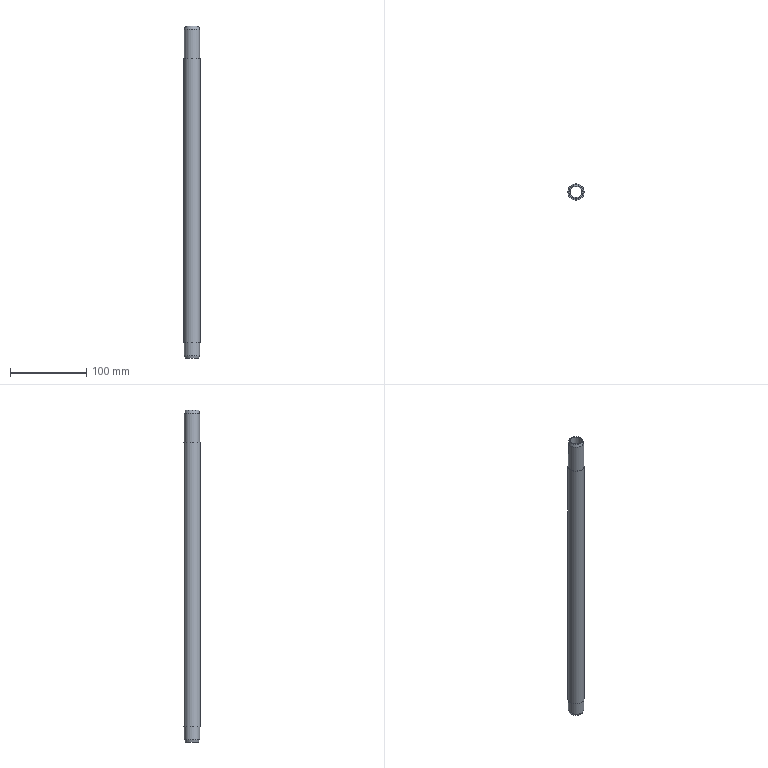Component | NX | CH3404_8-3 | 1 solid | 10 faces | box 21.3 x 21.3 x 435 mm | volume 75305 mm3 | plane 4 | cylinder 4 | cone 2 | commonest cylinder face diameters 20 x2 21.3 x1 15 x1
STEP:
#1=CARTESIAN_POINT('',(0.,0.,0.));
#2=DIRECTION('',(0.,0.,1.));
#3=DIRECTION('',(1.,0.,0.));
#4=AXIS2_PLACEMENT_3D('',#1,#2,#3);
#5=CARTESIAN_POINT('',(-10.65,0.,493.));
#6=VERTEX_POINT('',#5);
#7=CARTESIAN_POINT('',(0.,0.,493.));
#8=DIRECTION('',(0.,0.,-1.));
#9=DIRECTION('',(-1.,0.,0.));
#10=AXIS2_PLACEMENT_3D('',#7,#8,#9);
#11=CIRCLE('',#10,10.65);
#12=CARTESIAN_POINT('',(0.,-10.,493.));
#13=DIRECTION('',(0.,0.,-1.));
#14=DIRECTION('',(-1.,0.,0.));
#15=AXIS2_PLACEMENT_3D('',#12,#13,#14);
#16=PLANE('',#15);
#17=CARTESIAN_POINT('',(0.,10.));
#18=DIRECTION('',(1.,0.));
#19=AXIS2_PLACEMENT_2D('',#17,#18);
#20=CIRCLE('',#19,10.65);
#21=(GEOMETRIC_REPRESENTATION_CONTEXT(2)PARAMETRIC_REPRESENTATION_CONTEXT()REPRESENTATION_CONTEXT('',''));
#22=DEFINITIONAL_REPRESENTATION('',(#20),#21);
#23=PCURVE('',#16,#22);
#24=CARTESIAN_POINT('',(0.,0.,100.));
#25=DIRECTION('',(0.,0.,-1.));
#26=DIRECTION('',(-1.,0.,0.));
#27=AXIS2_PLACEMENT_3D('',#24,#25,#26);
#28=CYLINDRICAL_SURFACE('',#27,10.65);
#29=CARTESIAN_POINT('',(0.,-393.));
#30=DIRECTION('',(1.,0.));
#31=VECTOR('',#30,1.);
#32=LINE('',#29,#31);
#33=(GEOMETRIC_REPRESENTATION_CONTEXT(2)PARAMETRIC_REPRESENTATION_CONTEXT()REPRESENTATION_CONTEXT('',''));
#34=DEFINITIONAL_REPRESENTATION('',(#32),#33);
#35=PCURVE('',#28,#34);
#36=SURFACE_CURVE('',#11,(#23,#35),.PCURVE_S1.);
#37=EDGE_CURVE('',#6,#6,#36,.T.);
#38=ORIENTED_EDGE('',*,*,#37,.F.);
#39=EDGE_LOOP('',(#38));
#40=FACE_BOUND('',#39,.T.);
#41=CARTESIAN_POINT('',(-10.,0.,493.));
#42=VERTEX_POINT('',#41);
#43=CARTESIAN_POINT('',(0.,0.,493.));
#44=DIRECTION('',(0.,0.,-1.));
#45=DIRECTION('',(-1.,0.,0.));
#46=AXIS2_PLACEMENT_3D('',#43,#44,#45);
#47=CIRCLE('',#46,10.);
#48=CARTESIAN_POINT('',(0.,10.));
#49=DIRECTION('',(1.,0.));
#50=AXIS2_PLACEMENT_2D('',#48,#49);
#51=CIRCLE('',#50,10.);
#52=(GEOMETRIC_REPRESENTATION_CONTEXT(2)PARAMETRIC_REPRESENTATION_CONTEXT()REPRESENTATION_CONTEXT('',''));
#53=DEFINITIONAL_REPRESENTATION('',(#51),#52);
#54=PCURVE('',#16,#53);
#55=CARTESIAN_POINT('',(0.,0.,100.));
#56=DIRECTION('',(0.,0.,-1.));
#57=DIRECTION('',(-1.,0.,0.));
#58=AXIS2_PLACEMENT_3D('',#55,#56,#57);
#59=CYLINDRICAL_SURFACE('',#58,10.);
#60=CARTESIAN_POINT('',(0.,-393.));
#61=DIRECTION('',(1.,0.));
#62=VECTOR('',#61,1.);
#63=LINE('',#60,#62);
#64=(GEOMETRIC_REPRESENTATION_CONTEXT(2)PARAMETRIC_REPRESENTATION_CONTEXT()REPRESENTATION_CONTEXT('',''));
#65=DEFINITIONAL_REPRESENTATION('',(#63),#64);
#66=PCURVE('',#59,#65);
#67=SURFACE_CURVE('',#47,(#54,#66),.PCURVE_S1.);
#68=EDGE_CURVE('',#42,#42,#67,.T.);
#69=ORIENTED_EDGE('',*,*,#68,.T.);
#70=EDGE_LOOP('',(#69));
#71=FACE_BOUND('',#70,.T.);
#72=ADVANCED_FACE('',(#40,#71),#16,.F.);
#73=CARTESIAN_POINT('',(-10.65,0.,120.));
#74=VERTEX_POINT('',#73);
#75=CARTESIAN_POINT('',(0.,0.,120.));
#76=DIRECTION('',(0.,0.,-1.));
#77=DIRECTION('',(-1.,0.,0.));
#78=AXIS2_PLACEMENT_3D('',#75,#76,#77);
#79=CIRCLE('',#78,10.65);
#80=CARTESIAN_POINT('',(0.,-20.));
#81=DIRECTION('',(1.,0.));
#82=VECTOR('',#81,1.);
#83=LINE('',#80,#82);
#84=(GEOMETRIC_REPRESENTATION_CONTEXT(2)PARAMETRIC_REPRESENTATION_CONTEXT()REPRESENTATION_CONTEXT('',''));
#85=DEFINITIONAL_REPRESENTATION('',(#83),#84);
#86=PCURVE('',#28,#85);
#87=CARTESIAN_POINT('',(0.,-10.65,120.));
#88=DIRECTION('',(0.,0.,1.));
#89=DIRECTION('',(1.,0.,0.));
#90=AXIS2_PLACEMENT_3D('',#87,#88,#89);
#91=PLANE('',#90);
#92=CARTESIAN_POINT('',(-10.65,10.65));
#93=CARTESIAN_POINT('',(-10.65,29.096));
#94=CARTESIAN_POINT('',(5.325,19.873));
#95=CARTESIAN_POINT('',(21.3,10.65));
#96=CARTESIAN_POINT('',(5.325,1.427));
#97=CARTESIAN_POINT('',(-10.65,-7.796));
#98=CARTESIAN_POINT('',(-10.65,10.65));
#99=(BOUNDED_CURVE()B_SPLINE_CURVE(2,(#92,#93,#94,#95,#96,#97,#98),.UNSPECIFIED.,.T.,.F.)B_SPLINE_CURVE_WITH_KNOTS((1,2,2,2,2,1),(-2.094,0.,2.094,4.189,6.283,8.378),.UNSPECIFIED.)CURVE()GEOMETRIC_REPRESENTATION_ITEM()RATIONAL_B_SPLINE_CURVE((1.,0.5,1.,0.5,1.,0.5,1.))REPRESENTATION_ITEM(''));
#100=(GEOMETRIC_REPRESENTATION_CONTEXT(2)PARAMETRIC_REPRESENTATION_CONTEXT()REPRESENTATION_CONTEXT('',''));
#101=DEFINITIONAL_REPRESENTATION('',(#99),#100);
#102=PCURVE('',#91,#101);
#103=SURFACE_CURVE('',#79,(#86,#102),.PCURVE_S1.);
#104=EDGE_CURVE('',#74,#74,#103,.T.);
#105=ORIENTED_EDGE('',*,*,#104,.F.);
#106=CARTESIAN_POINT('',(-10.65,-0.,493.));
#107=CARTESIAN_POINT('',(-10.65,-0.,120.));
#108=B_SPLINE_CURVE_WITH_KNOTS('',1,(#106,#107),.UNSPECIFIED.,.F.,.F.,(2,2),(-393.,-20.),.PIECEWISE_BEZIER_KNOTS.);
#109=CARTESIAN_POINT('',(0.,0.));
#110=DIRECTION('',(0.,1.));
#111=VECTOR('',#110,1.);
#112=LINE('',#109,#111);
#113=(GEOMETRIC_REPRESENTATION_CONTEXT(2)PARAMETRIC_REPRESENTATION_CONTEXT()REPRESENTATION_CONTEXT('',''));
#114=DEFINITIONAL_REPRESENTATION('',(#112),#113);
#115=PCURVE('',#28,#114);
#116=CARTESIAN_POINT('',(6.283,0.));
#117=DIRECTION('',(0.,1.));
#118=VECTOR('',#117,1.);
#119=LINE('',#116,#118);
#120=(GEOMETRIC_REPRESENTATION_CONTEXT(2)PARAMETRIC_REPRESENTATION_CONTEXT()REPRESENTATION_CONTEXT('',''));
#121=DEFINITIONAL_REPRESENTATION('',(#119),#120);
#122=PCURVE('',#28,#121);
#123=SEAM_CURVE('',#108,(#115,#122),.PCURVE_S1.);
#124=EDGE_CURVE('',#6,#74,#123,.T.);
#125=ORIENTED_EDGE('',*,*,#124,.F.);
#126=ORIENTED_EDGE('',*,*,#37,.T.);
#127=ORIENTED_EDGE('',*,*,#124,.T.);
#128=EDGE_LOOP('',(#105,#125,#126,#127));
#129=FACE_BOUND('',#128,.T.);
#130=ADVANCED_FACE('',(#129),#28,.T.);
#131=CARTESIAN_POINT('',(-10.,0.,120.));
#132=VERTEX_POINT('',#131);
#133=CARTESIAN_POINT('',(0.,0.,120.));
#134=DIRECTION('',(0.,0.,-1.));
#135=DIRECTION('',(-1.,0.,0.));
#136=AXIS2_PLACEMENT_3D('',#133,#134,#135);
#137=CIRCLE('',#136,10.);
#138=CARTESIAN_POINT('',(-10.,10.65));
#139=CARTESIAN_POINT('',(-10.,27.971));
#140=CARTESIAN_POINT('',(5.,19.31));
#141=CARTESIAN_POINT('',(20.,10.65));
#142=CARTESIAN_POINT('',(5.,1.99));
#143=CARTESIAN_POINT('',(-10.,-6.671));
#144=CARTESIAN_POINT('',(-10.,10.65));
#145=(BOUNDED_CURVE()B_SPLINE_CURVE(2,(#138,#139,#140,#141,#142,#143,#144),.UNSPECIFIED.,.T.,.F.)B_SPLINE_CURVE_WITH_KNOTS((1,2,2,2,2,1),(-2.094,0.,2.094,4.189,6.283,8.378),.UNSPECIFIED.)CURVE()GEOMETRIC_REPRESENTATION_ITEM()RATIONAL_B_SPLINE_CURVE((1.,0.5,1.,0.5,1.,0.5,1.))REPRESENTATION_ITEM(''));
#146=(GEOMETRIC_REPRESENTATION_CONTEXT(2)PARAMETRIC_REPRESENTATION_CONTEXT()REPRESENTATION_CONTEXT('',''));
#147=DEFINITIONAL_REPRESENTATION('',(#145),#146);
#148=PCURVE('',#91,#147);
#149=CARTESIAN_POINT('',(0.,0.,100.));
#150=DIRECTION('',(0.,0.,-1.));
#151=DIRECTION('',(-1.,0.,0.));
#152=AXIS2_PLACEMENT_3D('',#149,#150,#151);
#153=CYLINDRICAL_SURFACE('',#152,10.);
#154=CARTESIAN_POINT('',(0.,-20.));
#155=DIRECTION('',(1.,0.));
#156=VECTOR('',#155,1.);
#157=LINE('',#154,#156);
#158=(GEOMETRIC_REPRESENTATION_CONTEXT(2)PARAMETRIC_REPRESENTATION_CONTEXT()REPRESENTATION_CONTEXT('',''));
#159=DEFINITIONAL_REPRESENTATION('',(#157),#158);
#160=PCURVE('',#153,#159);
#161=SURFACE_CURVE('',#137,(#148,#160),.PCURVE_S1.);
#162=EDGE_CURVE('',#132,#132,#161,.T.);
#163=ORIENTED_EDGE('',*,*,#162,.F.);
#164=EDGE_LOOP('',(#163));
#165=FACE_BOUND('',#164,.T.);
#166=ORIENTED_EDGE('',*,*,#104,.T.);
#167=EDGE_LOOP('',(#166));
#168=FACE_BOUND('',#167,.T.);
#169=ADVANCED_FACE('',(#165,#168),#91,.F.);
#170=CARTESIAN_POINT('',(10.,0.,103.));
#171=VERTEX_POINT('',#170);
#172=CARTESIAN_POINT('',(-10.,0.,103.));
#173=VERTEX_POINT('',#172);
#174=CARTESIAN_POINT('',(0.,0.,103.));
#175=DIRECTION('',(0.,0.,1.));
#176=DIRECTION('',(1.,0.,0.));
#177=AXIS2_PLACEMENT_3D('',#174,#175,#176);
#178=CIRCLE('',#177,10.);
#179=CARTESIAN_POINT('',(3.142,-3.));
#180=DIRECTION('',(-1.,0.));
#181=VECTOR('',#180,1.);
#182=LINE('',#179,#181);
#183=(GEOMETRIC_REPRESENTATION_CONTEXT(2)PARAMETRIC_REPRESENTATION_CONTEXT()REPRESENTATION_CONTEXT('',''));
#184=DEFINITIONAL_REPRESENTATION('',(#182),#183);
#185=PCURVE('',#153,#184);
#186=CARTESIAN_POINT('',(0.,0.,100.));
#187=DIRECTION('',(0.,0.,1.));
#188=DIRECTION('',(1.,0.,0.));
#189=AXIS2_PLACEMENT_3D('',#186,#187,#188);
#190=CONICAL_SURFACE('',#189,9.,0.3218);
#191=CARTESIAN_POINT('',(0.,3.));
#192=DIRECTION('',(1.,0.));
#193=VECTOR('',#192,1.);
#194=LINE('',#191,#193);
#195=(GEOMETRIC_REPRESENTATION_CONTEXT(2)PARAMETRIC_REPRESENTATION_CONTEXT()REPRESENTATION_CONTEXT('',''));
#196=DEFINITIONAL_REPRESENTATION('',(#194),#195);
#197=PCURVE('',#190,#196);
#198=SURFACE_CURVE('',#178,(#185,#197),.PCURVE_S1.);
#199=EDGE_CURVE('',#171,#173,#198,.T.);
#200=ORIENTED_EDGE('',*,*,#199,.T.);
#201=CARTESIAN_POINT('',(-10.,-0.,120.));
#202=CARTESIAN_POINT('',(-10.,-0.,103.));
#203=B_SPLINE_CURVE_WITH_KNOTS('',1,(#201,#202),.UNSPECIFIED.,.F.,.F.,(2,2),(-20.,-3.),.PIECEWISE_BEZIER_KNOTS.);
#204=CARTESIAN_POINT('',(0.,0.));
#205=DIRECTION('',(0.,1.));
#206=VECTOR('',#205,1.);
#207=LINE('',#204,#206);
#208=(GEOMETRIC_REPRESENTATION_CONTEXT(2)PARAMETRIC_REPRESENTATION_CONTEXT()REPRESENTATION_CONTEXT('',''));
#209=DEFINITIONAL_REPRESENTATION('',(#207),#208);
#210=PCURVE('',#153,#209);
#211=CARTESIAN_POINT('',(6.283,0.));
#212=DIRECTION('',(0.,1.));
#213=VECTOR('',#212,1.);
#214=LINE('',#211,#213);
#215=(GEOMETRIC_REPRESENTATION_CONTEXT(2)PARAMETRIC_REPRESENTATION_CONTEXT()REPRESENTATION_CONTEXT('',''));
#216=DEFINITIONAL_REPRESENTATION('',(#214),#215);
#217=PCURVE('',#153,#216);
#218=SEAM_CURVE('',#203,(#210,#217),.PCURVE_S1.);
#219=EDGE_CURVE('',#132,#173,#218,.T.);
#220=ORIENTED_EDGE('',*,*,#219,.F.);
#221=ORIENTED_EDGE('',*,*,#162,.T.);
#222=ORIENTED_EDGE('',*,*,#219,.T.);
#223=CARTESIAN_POINT('',(0.,0.,103.));
#224=DIRECTION('',(0.,0.,1.));
#225=DIRECTION('',(1.,0.,0.));
#226=AXIS2_PLACEMENT_3D('',#223,#224,#225);
#227=CIRCLE('',#226,10.);
#228=CARTESIAN_POINT('',(9.425,-3.));
#229=DIRECTION('',(-1.,0.));
#230=VECTOR('',#229,1.);
#231=LINE('',#228,#230);
#232=(GEOMETRIC_REPRESENTATION_CONTEXT(2)PARAMETRIC_REPRESENTATION_CONTEXT()REPRESENTATION_CONTEXT('',''));
#233=DEFINITIONAL_REPRESENTATION('',(#231),#232);
#234=PCURVE('',#153,#233);
#235=CARTESIAN_POINT('',(0.,3.));
#236=DIRECTION('',(1.,0.));
#237=VECTOR('',#236,1.);
#238=LINE('',#235,#237);
#239=(GEOMETRIC_REPRESENTATION_CONTEXT(2)PARAMETRIC_REPRESENTATION_CONTEXT()REPRESENTATION_CONTEXT('',''));
#240=DEFINITIONAL_REPRESENTATION('',(#238),#239);
#241=PCURVE('',#190,#240);
#242=SURFACE_CURVE('',#227,(#234,#241),.PCURVE_S1.);
#243=EDGE_CURVE('',#173,#171,#242,.T.);
#244=ORIENTED_EDGE('',*,*,#243,.T.);
#245=EDGE_LOOP('',(#200,#220,#221,#222,#244));
#246=FACE_BOUND('',#245,.T.);
#247=ADVANCED_FACE('',(#246),#153,.T.);
#248=CARTESIAN_POINT('',(9.,0.,100.));
#249=VERTEX_POINT('',#248);
#250=CARTESIAN_POINT('',(0.,0.,100.));
#251=DIRECTION('',(0.,0.,-1.));
#252=DIRECTION('',(1.,0.,0.));
#253=AXIS2_PLACEMENT_3D('',#250,#251,#252);
#254=CIRCLE('',#253,9.);
#255=CARTESIAN_POINT('',(0.,-10.,100.));
#256=DIRECTION('',(0.,0.,1.));
#257=DIRECTION('',(1.,0.,0.));
#258=AXIS2_PLACEMENT_3D('',#255,#256,#257);
#259=PLANE('',#258);
#260=CARTESIAN_POINT('',(9.,10.));
#261=CARTESIAN_POINT('',(9.,-5.588));
#262=CARTESIAN_POINT('',(-4.5,2.206));
#263=CARTESIAN_POINT('',(-18.,10.));
#264=CARTESIAN_POINT('',(-4.5,17.794));
#265=CARTESIAN_POINT('',(9.,25.588));
#266=CARTESIAN_POINT('',(9.,10.));
#267=(BOUNDED_CURVE()B_SPLINE_CURVE(2,(#260,#261,#262,#263,#264,#265,#266),.UNSPECIFIED.,.T.,.F.)B_SPLINE_CURVE_WITH_KNOTS((1,2,2,2,2,1),(-2.094,0.,2.094,4.189,6.283,8.378),.UNSPECIFIED.)CURVE()GEOMETRIC_REPRESENTATION_ITEM()RATIONAL_B_SPLINE_CURVE((1.,0.5,1.,0.5,1.,0.5,1.))REPRESENTATION_ITEM(''));
#268=(GEOMETRIC_REPRESENTATION_CONTEXT(2)PARAMETRIC_REPRESENTATION_CONTEXT()REPRESENTATION_CONTEXT('',''));
#269=DEFINITIONAL_REPRESENTATION('',(#267),#268);
#270=PCURVE('',#259,#269);
#271=CARTESIAN_POINT('',(6.283,0.));
#272=DIRECTION('',(-1.,0.));
#273=VECTOR('',#272,1.);
#274=LINE('',#271,#273);
#275=(GEOMETRIC_REPRESENTATION_CONTEXT(2)PARAMETRIC_REPRESENTATION_CONTEXT()REPRESENTATION_CONTEXT('',''));
#276=DEFINITIONAL_REPRESENTATION('',(#274),#275);
#277=PCURVE('',#190,#276);
#278=SURFACE_CURVE('',#254,(#270,#277),.PCURVE_S1.);
#279=EDGE_CURVE('',#249,#249,#278,.T.);
#280=ORIENTED_EDGE('',*,*,#279,.T.);
#281=EDGE_LOOP('',(#280));
#282=FACE_BOUND('',#281,.T.);
#283=CARTESIAN_POINT('',(-7.5,0.,100.));
#284=VERTEX_POINT('',#283);
#285=CARTESIAN_POINT('',(0.,0.,100.));
#286=DIRECTION('',(0.,0.,-1.));
#287=DIRECTION('',(-1.,0.,0.));
#288=AXIS2_PLACEMENT_3D('',#285,#286,#287);
#289=CIRCLE('',#288,7.5);
#290=CARTESIAN_POINT('',(-7.5,10.));
#291=CARTESIAN_POINT('',(-7.5,22.99));
#292=CARTESIAN_POINT('',(3.75,16.495));
#293=CARTESIAN_POINT('',(15.,10.));
#294=CARTESIAN_POINT('',(3.75,3.505));
#295=CARTESIAN_POINT('',(-7.5,-2.99));
#296=CARTESIAN_POINT('',(-7.5,10.));
#297=(BOUNDED_CURVE()B_SPLINE_CURVE(2,(#290,#291,#292,#293,#294,#295,#296),.UNSPECIFIED.,.T.,.F.)B_SPLINE_CURVE_WITH_KNOTS((1,2,2,2,2,1),(-2.094,0.,2.094,4.189,6.283,8.378),.UNSPECIFIED.)CURVE()GEOMETRIC_REPRESENTATION_ITEM()RATIONAL_B_SPLINE_CURVE((1.,0.5,1.,0.5,1.,0.5,1.))REPRESENTATION_ITEM(''));
#298=(GEOMETRIC_REPRESENTATION_CONTEXT(2)PARAMETRIC_REPRESENTATION_CONTEXT()REPRESENTATION_CONTEXT('',''));
#299=DEFINITIONAL_REPRESENTATION('',(#297),#298);
#300=PCURVE('',#259,#299);
#301=CARTESIAN_POINT('',(0.,0.,100.));
#302=DIRECTION('',(0.,0.,-1.));
#303=DIRECTION('',(-1.,0.,0.));
#304=AXIS2_PLACEMENT_3D('',#301,#302,#303);
#305=CYLINDRICAL_SURFACE('',#304,7.5);
#306=CARTESIAN_POINT('',(0.,0.));
#307=DIRECTION('',(1.,0.));
#308=VECTOR('',#307,1.);
#309=LINE('',#306,#308);
#310=(GEOMETRIC_REPRESENTATION_CONTEXT(2)PARAMETRIC_REPRESENTATION_CONTEXT()REPRESENTATION_CONTEXT('',''));
#311=DEFINITIONAL_REPRESENTATION('',(#309),#310);
#312=PCURVE('',#305,#311);
#313=SURFACE_CURVE('',#289,(#300,#312),.PCURVE_S1.);
#314=EDGE_CURVE('',#284,#284,#313,.T.);
#315=ORIENTED_EDGE('',*,*,#314,.F.);
#316=EDGE_LOOP('',(#315));
#317=FACE_BOUND('',#316,.T.);
#318=ADVANCED_FACE('',(#282,#317),#259,.F.);
#319=CARTESIAN_POINT('',(-7.5,0.,535.));
#320=VERTEX_POINT('',#319);
#321=CARTESIAN_POINT('',(0.,0.,535.));
#322=DIRECTION('',(0.,0.,-1.));
#323=DIRECTION('',(-1.,0.,0.));
#324=AXIS2_PLACEMENT_3D('',#321,#322,#323);
#325=CIRCLE('',#324,7.5);
#326=CARTESIAN_POINT('',(0.,-435.));
#327=DIRECTION('',(1.,0.));
#328=VECTOR('',#327,1.);
#329=LINE('',#326,#328);
#330=(GEOMETRIC_REPRESENTATION_CONTEXT(2)PARAMETRIC_REPRESENTATION_CONTEXT()REPRESENTATION_CONTEXT('',''));
#331=DEFINITIONAL_REPRESENTATION('',(#329),#330);
#332=PCURVE('',#305,#331);
#333=CARTESIAN_POINT('',(0.,-7.5,535.));
#334=DIRECTION('',(0.,0.,-1.));
#335=DIRECTION('',(-1.,0.,0.));
#336=AXIS2_PLACEMENT_3D('',#333,#334,#335);
#337=PLANE('',#336);
#338=CARTESIAN_POINT('',(0.,7.5));
#339=DIRECTION('',(1.,0.));
#340=AXIS2_PLACEMENT_2D('',#338,#339);
#341=CIRCLE('',#340,7.5);
#342=(GEOMETRIC_REPRESENTATION_CONTEXT(2)PARAMETRIC_REPRESENTATION_CONTEXT()REPRESENTATION_CONTEXT('',''));
#343=DEFINITIONAL_REPRESENTATION('',(#341),#342);
#344=PCURVE('',#337,#343);
#345=SURFACE_CURVE('',#325,(#332,#344),.PCURVE_S1.);
#346=EDGE_CURVE('',#320,#320,#345,.T.);
#347=ORIENTED_EDGE('',*,*,#346,.T.);
#348=CARTESIAN_POINT('',(-7.5,0.,535.));
#349=CARTESIAN_POINT('',(-7.5,0.,100.));
#350=B_SPLINE_CURVE_WITH_KNOTS('',1,(#348,#349),.UNSPECIFIED.,.F.,.F.,(2,2),(-435.,0.),.PIECEWISE_BEZIER_KNOTS.);
#351=CARTESIAN_POINT('',(6.283,0.));
#352=DIRECTION('',(0.,1.));
#353=VECTOR('',#352,1.);
#354=LINE('',#351,#353);
#355=(GEOMETRIC_REPRESENTATION_CONTEXT(2)PARAMETRIC_REPRESENTATION_CONTEXT()REPRESENTATION_CONTEXT('',''));
#356=DEFINITIONAL_REPRESENTATION('',(#354),#355);
#357=PCURVE('',#305,#356);
#358=CARTESIAN_POINT('',(0.,0.));
#359=DIRECTION('',(0.,1.));
#360=VECTOR('',#359,1.);
#361=LINE('',#358,#360);
#362=(GEOMETRIC_REPRESENTATION_CONTEXT(2)PARAMETRIC_REPRESENTATION_CONTEXT()REPRESENTATION_CONTEXT('',''));
#363=DEFINITIONAL_REPRESENTATION('',(#361),#362);
#364=PCURVE('',#305,#363);
#365=SEAM_CURVE('',#350,(#357,#364),.PCURVE_S1.);
#366=EDGE_CURVE('',#320,#284,#365,.T.);
#367=ORIENTED_EDGE('',*,*,#366,.T.);
#368=ORIENTED_EDGE('',*,*,#314,.F.);
#369=ORIENTED_EDGE('',*,*,#366,.F.);
#370=EDGE_LOOP('',(#347,#367,#368,#369));
#371=FACE_BOUND('',#370,.F.);
#372=ADVANCED_FACE('',(#371),#305,.F.);
#373=CARTESIAN_POINT('',(-9.,0.,535.));
#374=VERTEX_POINT('',#373);
#375=CARTESIAN_POINT('',(0.,0.,535.));
#376=DIRECTION('',(0.,0.,-1.));
#377=DIRECTION('',(-1.,0.,0.));
#378=AXIS2_PLACEMENT_3D('',#375,#376,#377);
#379=CIRCLE('',#378,9.);
#380=CARTESIAN_POINT('',(0.,7.5));
#381=DIRECTION('',(1.,0.));
#382=AXIS2_PLACEMENT_2D('',#380,#381);
#383=CIRCLE('',#382,9.);
#384=(GEOMETRIC_REPRESENTATION_CONTEXT(2)PARAMETRIC_REPRESENTATION_CONTEXT()REPRESENTATION_CONTEXT('',''));
#385=DEFINITIONAL_REPRESENTATION('',(#383),#384);
#386=PCURVE('',#337,#385);
#387=CARTESIAN_POINT('',(0.,0.,535.));
#388=DIRECTION('',(0.,0.,-1.));
#389=DIRECTION('',(-1.,0.,0.));
#390=AXIS2_PLACEMENT_3D('',#387,#388,#389);
#391=CONICAL_SURFACE('',#390,9.,0.245);
#392=CARTESIAN_POINT('',(0.,0.));
#393=DIRECTION('',(1.,0.));
#394=VECTOR('',#393,1.);
#395=LINE('',#392,#394);
#396=(GEOMETRIC_REPRESENTATION_CONTEXT(2)PARAMETRIC_REPRESENTATION_CONTEXT()REPRESENTATION_CONTEXT('',''));
#397=DEFINITIONAL_REPRESENTATION('',(#395),#396);
#398=PCURVE('',#391,#397);
#399=SURFACE_CURVE('',#379,(#386,#398),.PCURVE_S1.);
#400=EDGE_CURVE('',#374,#374,#399,.T.);
#401=ORIENTED_EDGE('',*,*,#400,.F.);
#402=EDGE_LOOP('',(#401));
#403=FACE_BOUND('',#402,.T.);
#404=ORIENTED_EDGE('',*,*,#346,.T.);
#405=EDGE_LOOP('',(#404));
#406=FACE_BOUND('',#405,.T.);
#407=ADVANCED_FACE('',(#403,#406),#337,.F.);
#408=CARTESIAN_POINT('',(-10.,0.,531.));
#409=VERTEX_POINT('',#408);
#410=CARTESIAN_POINT('',(0.,0.,531.));
#411=DIRECTION('',(0.,0.,-1.));
#412=DIRECTION('',(-1.,0.,0.));
#413=AXIS2_PLACEMENT_3D('',#410,#411,#412);
#414=CIRCLE('',#413,10.);
#415=CARTESIAN_POINT('',(0.,4.));
#416=DIRECTION('',(1.,0.));
#417=VECTOR('',#416,1.);
#418=LINE('',#415,#417);
#419=(GEOMETRIC_REPRESENTATION_CONTEXT(2)PARAMETRIC_REPRESENTATION_CONTEXT()REPRESENTATION_CONTEXT('',''));
#420=DEFINITIONAL_REPRESENTATION('',(#418),#419);
#421=PCURVE('',#391,#420);
#422=CARTESIAN_POINT('',(0.,-431.));
#423=DIRECTION('',(1.,0.));
#424=VECTOR('',#423,1.);
#425=LINE('',#422,#424);
#426=(GEOMETRIC_REPRESENTATION_CONTEXT(2)PARAMETRIC_REPRESENTATION_CONTEXT()REPRESENTATION_CONTEXT('',''));
#427=DEFINITIONAL_REPRESENTATION('',(#425),#426);
#428=PCURVE('',#59,#427);
#429=SURFACE_CURVE('',#414,(#421,#428),.PCURVE_S1.);
#430=EDGE_CURVE('',#409,#409,#429,.T.);
#431=ORIENTED_EDGE('',*,*,#430,.F.);
#432=CARTESIAN_POINT('',(-9.,-0.,535.));
#433=CARTESIAN_POINT('',(-10.,-0.,531.));
#434=B_SPLINE_CURVE_WITH_KNOTS('',1,(#432,#433),.UNSPECIFIED.,.F.,.F.,(2,2),(0.,4.123),.PIECEWISE_BEZIER_KNOTS.);
#435=CARTESIAN_POINT('',(0.,0.));
#436=DIRECTION('',(0.,1.));
#437=VECTOR('',#436,1.);
#438=LINE('',#435,#437);
#439=(GEOMETRIC_REPRESENTATION_CONTEXT(2)PARAMETRIC_REPRESENTATION_CONTEXT()REPRESENTATION_CONTEXT('',''));
#440=DEFINITIONAL_REPRESENTATION('',(#438),#439);
#441=PCURVE('',#391,#440);
#442=CARTESIAN_POINT('',(6.283,0.));
#443=DIRECTION('',(0.,1.));
#444=VECTOR('',#443,1.);
#445=LINE('',#442,#444);
#446=(GEOMETRIC_REPRESENTATION_CONTEXT(2)PARAMETRIC_REPRESENTATION_CONTEXT()REPRESENTATION_CONTEXT('',''));
#447=DEFINITIONAL_REPRESENTATION('',(#445),#446);
#448=PCURVE('',#391,#447);
#449=SEAM_CURVE('',#434,(#441,#448),.PCURVE_S1.);
#450=EDGE_CURVE('',#374,#409,#449,.T.);
#451=ORIENTED_EDGE('',*,*,#450,.F.);
#452=ORIENTED_EDGE('',*,*,#400,.T.);
#453=ORIENTED_EDGE('',*,*,#450,.T.);
#454=EDGE_LOOP('',(#431,#451,#452,#453));
#455=FACE_BOUND('',#454,.T.);
#456=ADVANCED_FACE('',(#455),#391,.T.);
#457=ORIENTED_EDGE('',*,*,#68,.F.);
#458=CARTESIAN_POINT('',(-10.,-0.,531.));
#459=CARTESIAN_POINT('',(-10.,-0.,493.));
#460=B_SPLINE_CURVE_WITH_KNOTS('',1,(#458,#459),.UNSPECIFIED.,.F.,.F.,(2,2),(-431.,-393.),.PIECEWISE_BEZIER_KNOTS.);
#461=CARTESIAN_POINT('',(0.,0.));
#462=DIRECTION('',(0.,1.));
#463=VECTOR('',#462,1.);
#464=LINE('',#461,#463);
#465=(GEOMETRIC_REPRESENTATION_CONTEXT(2)PARAMETRIC_REPRESENTATION_CONTEXT()REPRESENTATION_CONTEXT('',''));
#466=DEFINITIONAL_REPRESENTATION('',(#464),#465);
#467=PCURVE('',#59,#466);
#468=CARTESIAN_POINT('',(6.283,0.));
#469=DIRECTION('',(0.,1.));
#470=VECTOR('',#469,1.);
#471=LINE('',#468,#470);
#472=(GEOMETRIC_REPRESENTATION_CONTEXT(2)PARAMETRIC_REPRESENTATION_CONTEXT()REPRESENTATION_CONTEXT('',''));
#473=DEFINITIONAL_REPRESENTATION('',(#471),#472);
#474=PCURVE('',#59,#473);
#475=SEAM_CURVE('',#460,(#467,#474),.PCURVE_S1.);
#476=EDGE_CURVE('',#409,#42,#475,.T.);
#477=ORIENTED_EDGE('',*,*,#476,.F.);
#478=ORIENTED_EDGE('',*,*,#430,.T.);
#479=ORIENTED_EDGE('',*,*,#476,.T.);
#480=EDGE_LOOP('',(#457,#477,#478,#479));
#481=FACE_BOUND('',#480,.T.);
#482=ADVANCED_FACE('',(#481),#59,.T.);
#483=ORIENTED_EDGE('',*,*,#199,.F.);
#484=CARTESIAN_POINT('',(9.,-0.,100.));
#485=CARTESIAN_POINT('',(10.,-0.,103.));
#486=B_SPLINE_CURVE_WITH_KNOTS('',1,(#484,#485),.UNSPECIFIED.,.F.,.F.,(2,2),(0.,3.162),.PIECEWISE_BEZIER_KNOTS.);
#487=CARTESIAN_POINT('',(0.,0.));
#488=DIRECTION('',(0.,1.));
#489=VECTOR('',#488,1.);
#490=LINE('',#487,#489);
#491=(GEOMETRIC_REPRESENTATION_CONTEXT(2)PARAMETRIC_REPRESENTATION_CONTEXT()REPRESENTATION_CONTEXT('',''));
#492=DEFINITIONAL_REPRESENTATION('',(#490),#491);
#493=PCURVE('',#190,#492);
#494=CARTESIAN_POINT('',(6.283,0.));
#495=DIRECTION('',(0.,1.));
#496=VECTOR('',#495,1.);
#497=LINE('',#494,#496);
#498=(GEOMETRIC_REPRESENTATION_CONTEXT(2)PARAMETRIC_REPRESENTATION_CONTEXT()REPRESENTATION_CONTEXT('',''));
#499=DEFINITIONAL_REPRESENTATION('',(#497),#498);
#500=PCURVE('',#190,#499);
#501=SEAM_CURVE('',#486,(#493,#500),.PCURVE_S1.);
#502=EDGE_CURVE('',#249,#171,#501,.T.);
#503=ORIENTED_EDGE('',*,*,#502,.F.);
#504=ORIENTED_EDGE('',*,*,#279,.F.);
#505=ORIENTED_EDGE('',*,*,#502,.T.);
#506=ORIENTED_EDGE('',*,*,#243,.F.);
#507=EDGE_LOOP('',(#483,#503,#504,#505,#506));
#508=FACE_BOUND('',#507,.T.);
#509=ADVANCED_FACE('',(#508),#190,.T.);
#510=CLOSED_SHELL('',(#72,#130,#169,#247,#318,#372,#407,#456,#482,#509));
#511=MANIFOLD_SOLID_BREP('',#510);
#512=(LENGTH_UNIT()NAMED_UNIT(*)SI_UNIT(.MILLI.,.METRE.));
#513=UNCERTAINTY_MEASURE_WITH_UNIT(LENGTH_MEASURE(0.00001),#512,'','');
#514=(NAMED_UNIT(*)PLANE_ANGLE_UNIT()SI_UNIT($,.RADIAN.));
#515=(NAMED_UNIT(*)SI_UNIT($,.STERADIAN.)SOLID_ANGLE_UNIT());
#516=(GEOMETRIC_REPRESENTATION_CONTEXT(3)GLOBAL_UNCERTAINTY_ASSIGNED_CONTEXT((#513))GLOBAL_UNIT_ASSIGNED_CONTEXT((#512,#514,#515))REPRESENTATION_CONTEXT('',''));
#517=ADVANCED_BREP_SHAPE_REPRESENTATION('',(#4,#511),#516);